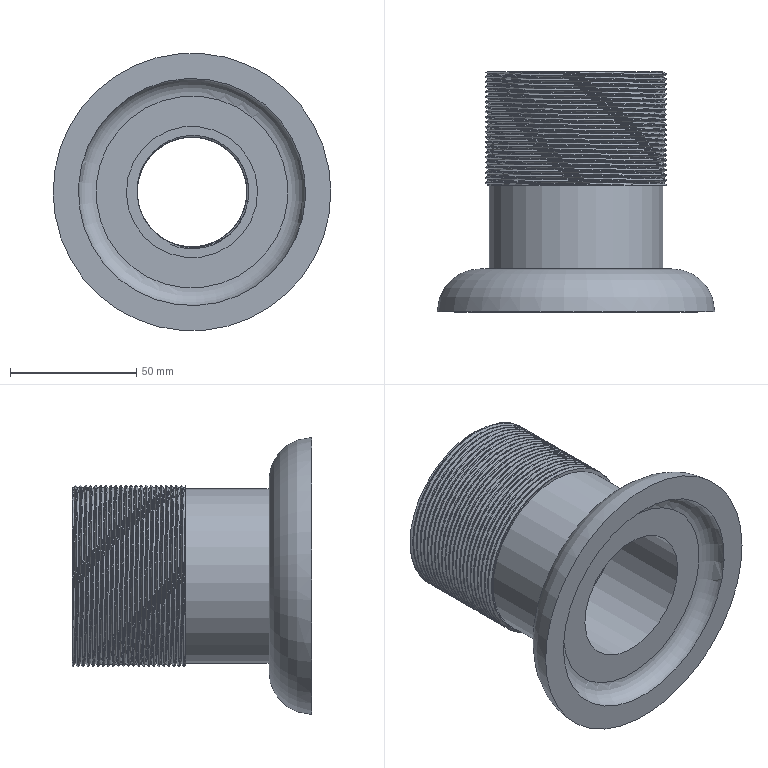Component | NX | SCREW_SLEEVE | 1 solid | 18 faces | volume 242809 mm3 | plane 6 | cylinder 6 | spline 4 | torus 2 | commonest cylinder face diameters 52 x1 43.5 x1 72 x1 69 x1 70 x1 45 x1